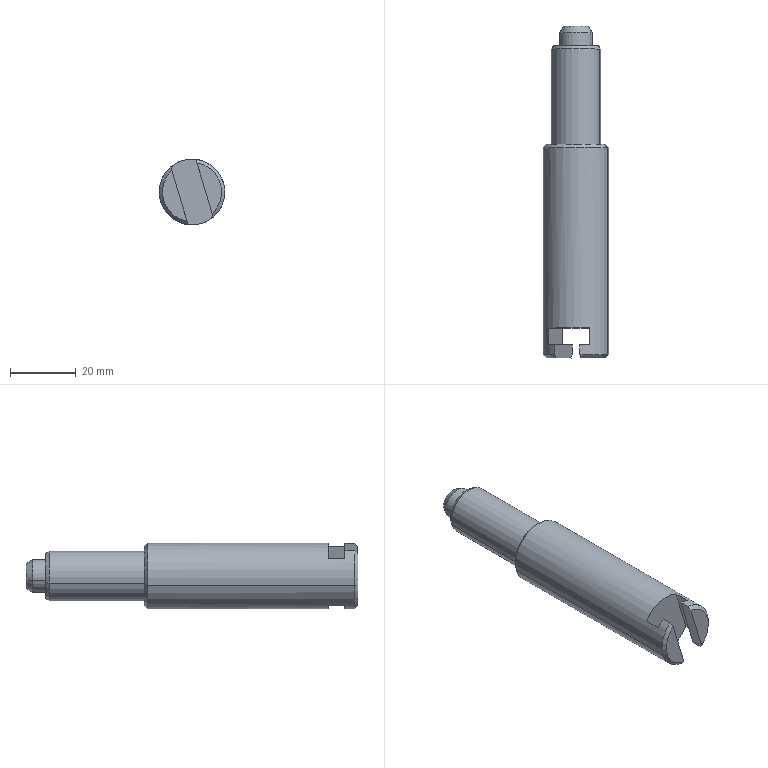Component | SolidWorks | BearingLiftingModule-1_CylinderLiftingModule-1_CHEN123-AA-27-1 | 1 solid | 27 faces | box 20 x 101 x 20 mm | volume 24230 mm3 | plane 12 | cone 9 | cylinder 6 | commonest cylinder face diameters 10 x2 15 x2 20 x2
build123d program:
from build123d import *

# Parameters (mm, degrees)
SKETCH1_R               = 10
BOSS_EXTRUDE1_DEPTH     = 65
SKETCH2_R               = 7.5
BOSS_EXTRUDE2_DEPTH     = 30
CHAMFER1_SIZE           = 1
CHAMFER1_SIZE2          = 0.5774
CHAMFER2_SIZE           = 1
CUT_EXTRUDE1_DEPTH      = 97.047
CUT_EXTRUDE1_DEPTH_BACK = 97.047
SKETCH4_R               = 5
BOSS_EXTRUDE3_DEPTH     = 6
CHAMFER3_SIZE           = 2
CHAMFER3_SIZE2          = 1.155


with BuildPart() as part:
    # Sketch1 → Boss-Extrude1 (new body)
    with BuildSketch(Plane.XY):
        Circle(SKETCH1_R)
    extrude(amount=BOSS_EXTRUDE1_DEPTH)

    # Sketch2 → Boss-Extrude2 (add)
    with BuildSketch(Plane.XY.offset(65)):
        Circle(SKETCH2_R)
    extrude(amount=BOSS_EXTRUDE2_DEPTH)

    # Chamfer1
    chamfer1_edges = [part.edges().sort_by_distance(p)[0] for p in [
        (-7.5, 0, 95),
    ]]
    chamfer1_side = [part.faces().sort_by_distance(p)[0] for p in [
        (-7.5, 0, 80),
    ]]
    chamfer(chamfer1_edges, length=CHAMFER1_SIZE, length2=CHAMFER1_SIZE2, reference=chamfer1_side[0])

    # Chamfer2
    chamfer2_edges = [part.edges().sort_by_distance(p)[0] for p in [
        (-10, 0, 0),
        (-10, 0, 65),
    ]]
    chamfer(chamfer2_edges, length=CHAMFER2_SIZE)

    # Sketch3 → Cut-Extrude1 (cut, two sides: drawn at the far end of the back side and taken through both)
    with BuildSketch(Plane(origin=(0, 0, 0), x_dir=(1, 0, 0), z_dir=(0, 1, 0)).offset(-CUT_EXTRUDE1_DEPTH_BACK)):
        Polygon((-6.6, -4), (-6.6, -9.1), (6.6, -9.1), (6.6, -4), (4, -4), (4, 0), (-4, 0), (-4, -4), align=None)
    extrude(amount=CUT_EXTRUDE1_DEPTH + CUT_EXTRUDE1_DEPTH_BACK, mode=Mode.SUBTRACT)

    # Sketch4 → Boss-Extrude3 (add)
    with BuildSketch(Plane.XY.offset(95)):
        Circle(SKETCH4_R)
    extrude(amount=BOSS_EXTRUDE3_DEPTH)

    # Chamfer3
    chamfer3_edges = [part.edges().sort_by_distance(p)[0] for p in [
        (-5, 0, 101),
    ]]
    chamfer3_side = [part.faces().sort_by_distance(p)[0] for p in [
        (-5, 0, 98),
    ]]
    chamfer(chamfer3_edges, length=CHAMFER3_SIZE, length2=CHAMFER3_SIZE2, reference=chamfer3_side[0])


solid = part.part

# Placed as in the assembly
solid = solid.moved(Location((69.999, -44.699, 30), (-90, 0, 163.304)))
STEP:
#1=COLOUR_RGB('',0.7922,0.8196,0.9333);
#2=FILL_AREA_STYLE_COLOUR('',#1);
#3=FILL_AREA_STYLE('',(#2));
#4=SURFACE_STYLE_FILL_AREA(#3);
#5=SURFACE_SIDE_STYLE('',(#4));
#6=SURFACE_STYLE_USAGE(.BOTH.,#5);
#7=PRESENTATION_STYLE_ASSIGNMENT((#6));
#8=CARTESIAN_POINT('',(2.611,2.217,1.138));
#9=VERTEX_POINT('',#8);
#10=CARTESIAN_POINT('',(2.901,2.217,1.225));
#11=VERTEX_POINT('',#10);
#12=CARTESIAN_POINT('',(2.756,2.217,1.181));
#13=DIRECTION('',(-0.,1.,-0.));
#14=DIRECTION('',(-0.9578,0.,-0.2873));
#15=AXIS2_PLACEMENT_3D('',#12,#13,#14);
#16=CIRCLE('',#15,0.1514);
#17=EDGE_CURVE('',#9,#11,#16,.T.);
#18=ORIENTED_EDGE('',*,*,#17,.F.);
#19=CARTESIAN_POINT('',(2.567,2.138,1.125));
#20=VERTEX_POINT('',#19);
#21=CARTESIAN_POINT('',(2.611,2.217,1.138));
#22=DIRECTION('',(-0.4789,-0.866,-0.1436));
#23=VECTOR('',#22,39.37);
#24=LINE('',#21,#23);
#25=EDGE_CURVE('',#9,#20,#24,.T.);
#26=ORIENTED_EDGE('',*,*,#25,.T.);
#27=CARTESIAN_POINT('',(2.944,2.138,1.238));
#28=VERTEX_POINT('',#27);
#29=CARTESIAN_POINT('',(2.756,2.138,1.181));
#30=DIRECTION('',(0.,-1.,0.));
#31=DIRECTION('',(-0.9578,0.,-0.2873));
#32=AXIS2_PLACEMENT_3D('',#29,#30,#31);
#33=CIRCLE('',#32,0.1969);
#34=EDGE_CURVE('',#28,#20,#33,.T.);
#35=ORIENTED_EDGE('',*,*,#34,.F.);
#36=CARTESIAN_POINT('',(2.901,2.217,1.225));
#37=DIRECTION('',(0.4789,-0.866,0.1436));
#38=VECTOR('',#37,39.37);
#39=LINE('',#36,#38);
#40=EDGE_CURVE('',#11,#28,#39,.T.);
#41=ORIENTED_EDGE('',*,*,#40,.F.);
#42=EDGE_LOOP('',(#18,#26,#35,#41));
#43=FACE_OUTER_BOUND('',#42,.T.);
#44=CARTESIAN_POINT('',(2.756,2.217,1.181));
#45=DIRECTION('',(0.,-1.,0.));
#46=DIRECTION('',(0.9578,0.,0.2873));
#47=AXIS2_PLACEMENT_3D('',#44,#45,#46);
#48=CONICAL_SURFACE('',#47,0.1514,0.5236);
#49=ADVANCED_FACE('',(#43),#48,.T.);
#50=ORIENTED_EDGE('',*,*,#34,.T.);
#51=CARTESIAN_POINT('',(2.567,1.98,1.125));
#52=VERTEX_POINT('',#51);
#53=CARTESIAN_POINT('',(2.567,2.217,1.125));
#54=DIRECTION('',(0.,-1.,0.));
#55=VECTOR('',#54,39.37);
#56=LINE('',#53,#55);
#57=EDGE_CURVE('',#20,#52,#56,.T.);
#58=ORIENTED_EDGE('',*,*,#57,.T.);
#59=CARTESIAN_POINT('',(2.944,1.98,1.238));
#60=VERTEX_POINT('',#59);
#61=CARTESIAN_POINT('',(2.756,1.98,1.181));
#62=DIRECTION('',(-0.,1.,-0.));
#63=DIRECTION('',(-0.9578,0.,-0.2873));
#64=AXIS2_PLACEMENT_3D('',#61,#62,#63);
#65=CIRCLE('',#64,0.1969);
#66=EDGE_CURVE('',#52,#60,#65,.T.);
#67=ORIENTED_EDGE('',*,*,#66,.T.);
#68=CARTESIAN_POINT('',(2.944,2.217,1.238));
#69=DIRECTION('',(0.,-1.,0.));
#70=VECTOR('',#69,39.37);
#71=LINE('',#68,#70);
#72=EDGE_CURVE('',#28,#60,#71,.T.);
#73=ORIENTED_EDGE('',*,*,#72,.F.);
#74=EDGE_LOOP('',(#50,#58,#67,#73));
#75=FACE_OUTER_BOUND('',#74,.T.);
#76=CARTESIAN_POINT('',(2.756,2.217,1.181));
#77=DIRECTION('',(0.,-1.,0.));
#78=DIRECTION('',(0.9578,0.,0.2873));
#79=AXIS2_PLACEMENT_3D('',#76,#77,#78);
#80=CYLINDRICAL_SURFACE('',#79,0.1969);
#81=ADVANCED_FACE('',(#75),#80,.T.);
#82=CARTESIAN_POINT('',(2.416,0.7992,1.079));
#83=VERTEX_POINT('',#82);
#84=CARTESIAN_POINT('',(3.095,0.7992,1.283));
#85=VERTEX_POINT('',#84);
#86=CARTESIAN_POINT('',(2.756,0.7992,1.181));
#87=DIRECTION('',(-0.,1.,-0.));
#88=DIRECTION('',(-0.9578,0.,-0.2873));
#89=AXIS2_PLACEMENT_3D('',#86,#87,#88);
#90=CIRCLE('',#89,0.3543);
#91=EDGE_CURVE('',#83,#85,#90,.T.);
#92=ORIENTED_EDGE('',*,*,#91,.F.);
#93=CARTESIAN_POINT('',(2.379,0.7599,1.068));
#94=VERTEX_POINT('',#93);
#95=CARTESIAN_POINT('',(2.416,0.7992,1.079));
#96=DIRECTION('',(-0.6773,-0.7071,-0.2031));
#97=VECTOR('',#96,39.37);
#98=LINE('',#95,#97);
#99=EDGE_CURVE('',#83,#94,#98,.T.);
#100=ORIENTED_EDGE('',*,*,#99,.T.);
#101=CARTESIAN_POINT('',(3.133,0.7599,1.294));
#102=VERTEX_POINT('',#101);
#103=CARTESIAN_POINT('',(2.756,0.7599,1.181));
#104=DIRECTION('',(0.,-1.,0.));
#105=DIRECTION('',(-0.9578,0.,-0.2873));
#106=AXIS2_PLACEMENT_3D('',#103,#104,#105);
#107=CIRCLE('',#106,0.3937);
#108=EDGE_CURVE('',#102,#94,#107,.T.);
#109=ORIENTED_EDGE('',*,*,#108,.F.);
#110=CARTESIAN_POINT('',(3.095,0.7992,1.283));
#111=DIRECTION('',(0.6773,-0.7071,0.2031));
#112=VECTOR('',#111,39.37);
#113=LINE('',#110,#112);
#114=EDGE_CURVE('',#85,#102,#113,.T.);
#115=ORIENTED_EDGE('',*,*,#114,.F.);
#116=EDGE_LOOP('',(#92,#100,#109,#115));
#117=FACE_OUTER_BOUND('',#116,.T.);
#118=CARTESIAN_POINT('',(2.756,0.7992,1.181));
#119=DIRECTION('',(0.,-1.,0.));
#120=DIRECTION('',(0.9578,0.,0.2873));
#121=AXIS2_PLACEMENT_3D('',#118,#119,#120);
#122=CONICAL_SURFACE('',#121,0.3543,0.7854);
#123=ADVANCED_FACE('',(#117),#122,.T.);
#124=CARTESIAN_POINT('',(2.416,-1.76,1.079));
#125=VERTEX_POINT('',#124);
#126=CARTESIAN_POINT('',(2.696,-1.76,0.8318));
#127=VERTEX_POINT('',#126);
#128=CARTESIAN_POINT('',(2.756,-1.76,1.181));
#129=DIRECTION('',(0.,-1.,0.));
#130=DIRECTION('',(-0.9578,0.,-0.2873));
#131=AXIS2_PLACEMENT_3D('',#128,#129,#130);
#132=CIRCLE('',#131,0.3543);
#133=EDGE_CURVE('',#125,#127,#132,.T.);
#134=ORIENTED_EDGE('',*,*,#133,.F.);
#135=CARTESIAN_POINT('',(2.379,-1.72,1.068));
#136=VERTEX_POINT('',#135);
#137=CARTESIAN_POINT('',(2.379,-1.72,1.068));
#138=DIRECTION('',(-0.6773,0.7071,-0.2031));
#139=VECTOR('',#138,39.37);
#140=LINE('',#137,#139);
#141=EDGE_CURVE('',#125,#136,#140,.T.);
#142=ORIENTED_EDGE('',*,*,#141,.T.);
#143=CARTESIAN_POINT('',(2.709,-1.72,0.7902));
#144=VERTEX_POINT('',#143);
#145=CARTESIAN_POINT('',(2.756,-1.72,1.181));
#146=DIRECTION('',(-0.,1.,-0.));
#147=DIRECTION('',(-0.9578,0.,-0.2873));
#148=AXIS2_PLACEMENT_3D('',#145,#146,#147);
#149=CIRCLE('',#148,0.3937);
#150=EDGE_CURVE('',#144,#136,#149,.T.);
#151=ORIENTED_EDGE('',*,*,#150,.F.);
#152=CARTESIAN_POINT('',(2.696,-1.76,0.8318));
#153=CARTESIAN_POINT('',(2.7,-1.747,0.8179));
#154=CARTESIAN_POINT('',(2.705,-1.734,0.804));
#155=CARTESIAN_POINT('',(2.709,-1.72,0.7902));
#156=B_SPLINE_CURVE_WITH_KNOTS('',3,(#152,#153,#154,#155),.UNSPECIFIED.,.F.,.F.,(4,4),(0.03786,0.03933),.UNSPECIFIED.);
#157=EDGE_CURVE('',#127,#144,#156,.T.);
#158=ORIENTED_EDGE('',*,*,#157,.F.);
#159=EDGE_LOOP('',(#134,#142,#151,#158));
#160=FACE_OUTER_BOUND('',#159,.T.);
#161=CARTESIAN_POINT('',(2.756,-1.72,1.181));
#162=DIRECTION('',(-0.,1.,-0.));
#163=DIRECTION('',(-0.9578,0.,-0.2873));
#164=AXIS2_PLACEMENT_3D('',#161,#162,#163);
#165=CONICAL_SURFACE('',#164,0.3937,0.7854);
#166=ADVANCED_FACE('',(#160),#165,.T.);
#167=CARTESIAN_POINT('',(2.495,1.98,1.103));
#168=VERTEX_POINT('',#167);
#169=CARTESIAN_POINT('',(3.017,1.98,1.259));
#170=VERTEX_POINT('',#169);
#171=CARTESIAN_POINT('',(2.756,1.98,1.181));
#172=DIRECTION('',(-0.,1.,-0.));
#173=DIRECTION('',(-0.9578,0.,-0.2873));
#174=AXIS2_PLACEMENT_3D('',#171,#172,#173);
#175=CIRCLE('',#174,0.2725);
#176=EDGE_CURVE('',#168,#170,#175,.T.);
#177=ORIENTED_EDGE('',*,*,#176,.F.);
#178=CARTESIAN_POINT('',(2.473,1.941,1.096));
#179=VERTEX_POINT('',#178);
#180=CARTESIAN_POINT('',(2.495,1.98,1.103));
#181=DIRECTION('',(-0.4789,-0.866,-0.1436));
#182=VECTOR('',#181,39.37);
#183=LINE('',#180,#182);
#184=EDGE_CURVE('',#168,#179,#183,.T.);
#185=ORIENTED_EDGE('',*,*,#184,.T.);
#186=CARTESIAN_POINT('',(3.039,1.941,1.266));
#187=VERTEX_POINT('',#186);
#188=CARTESIAN_POINT('',(2.756,1.941,1.181));
#189=DIRECTION('',(0.,-1.,0.));
#190=DIRECTION('',(-0.9578,0.,-0.2873));
#191=AXIS2_PLACEMENT_3D('',#188,#189,#190);
#192=CIRCLE('',#191,0.2953);
#193=EDGE_CURVE('',#187,#179,#192,.T.);
#194=ORIENTED_EDGE('',*,*,#193,.F.);
#195=CARTESIAN_POINT('',(3.017,1.98,1.259));
#196=DIRECTION('',(0.4789,-0.866,0.1436));
#197=VECTOR('',#196,39.37);
#198=LINE('',#195,#197);
#199=EDGE_CURVE('',#170,#187,#198,.T.);
#200=ORIENTED_EDGE('',*,*,#199,.F.);
#201=EDGE_LOOP('',(#177,#185,#194,#200));
#202=FACE_OUTER_BOUND('',#201,.T.);
#203=CARTESIAN_POINT('',(2.756,1.98,1.181));
#204=DIRECTION('',(0.,-1.,0.));
#205=DIRECTION('',(0.9578,0.,0.2873));
#206=AXIS2_PLACEMENT_3D('',#203,#204,#205);
#207=CONICAL_SURFACE('',#206,0.2725,0.5236);
#208=ADVANCED_FACE('',(#202),#207,.T.);
#209=ORIENTED_EDGE('',*,*,#193,.T.);
#210=CARTESIAN_POINT('',(2.473,0.7992,1.096));
#211=VERTEX_POINT('',#210);
#212=CARTESIAN_POINT('',(2.473,1.98,1.096));
#213=DIRECTION('',(0.,-1.,0.));
#214=VECTOR('',#213,39.37);
#215=LINE('',#212,#214);
#216=EDGE_CURVE('',#179,#211,#215,.T.);
#217=ORIENTED_EDGE('',*,*,#216,.T.);
#218=CARTESIAN_POINT('',(3.039,0.7992,1.266));
#219=VERTEX_POINT('',#218);
#220=CARTESIAN_POINT('',(2.756,0.7992,1.181));
#221=DIRECTION('',(-0.,1.,-0.));
#222=DIRECTION('',(-0.9578,0.,-0.2873));
#223=AXIS2_PLACEMENT_3D('',#220,#221,#222);
#224=CIRCLE('',#223,0.2953);
#225=EDGE_CURVE('',#211,#219,#224,.T.);
#226=ORIENTED_EDGE('',*,*,#225,.T.);
#227=CARTESIAN_POINT('',(3.039,1.98,1.266));
#228=DIRECTION('',(0.,-1.,0.));
#229=VECTOR('',#228,39.37);
#230=LINE('',#227,#229);
#231=EDGE_CURVE('',#187,#219,#230,.T.);
#232=ORIENTED_EDGE('',*,*,#231,.F.);
#233=EDGE_LOOP('',(#209,#217,#226,#232));
#234=FACE_OUTER_BOUND('',#233,.T.);
#235=CARTESIAN_POINT('',(2.756,1.98,1.181));
#236=DIRECTION('',(0.,-1.,0.));
#237=DIRECTION('',(0.9578,0.,0.2873));
#238=AXIS2_PLACEMENT_3D('',#235,#236,#237);
#239=CYLINDRICAL_SURFACE('',#238,0.2953);
#240=ADVANCED_FACE('',(#234),#239,.T.);
#241=ORIENTED_EDGE('',*,*,#108,.T.);
#242=CARTESIAN_POINT('',(2.379,0.7992,1.068));
#243=DIRECTION('',(0.,-1.,0.));
#244=VECTOR('',#243,39.37);
#245=LINE('',#242,#244);
#246=EDGE_CURVE('',#94,#136,#245,.T.);
#247=ORIENTED_EDGE('',*,*,#246,.T.);
#248=CARTESIAN_POINT('',(2.501,-1.72,1.481));
#249=VERTEX_POINT('',#248);
#250=CARTESIAN_POINT('',(2.756,-1.72,1.181));
#251=DIRECTION('',(-0.,1.,-0.));
#252=DIRECTION('',(-0.9578,0.,-0.2873));
#253=AXIS2_PLACEMENT_3D('',#250,#251,#252);
#254=CIRCLE('',#253,0.3937);
#255=EDGE_CURVE('',#136,#249,#254,.T.);
#256=ORIENTED_EDGE('',*,*,#255,.T.);
#257=CARTESIAN_POINT('',(2.501,-1.602,1.481));
#258=VERTEX_POINT('',#257);
#259=CARTESIAN_POINT('',(2.501,0.7992,1.481));
#260=DIRECTION('',(-0.,1.,-0.));
#261=VECTOR('',#260,39.37);
#262=LINE('',#259,#261);
#263=EDGE_CURVE('',#249,#258,#262,.T.);
#264=ORIENTED_EDGE('',*,*,#263,.T.);
#265=CARTESIAN_POINT('',(2.422,-1.602,1.39));
#266=VERTEX_POINT('',#265);
#267=CARTESIAN_POINT('',(2.756,-1.602,1.181));
#268=DIRECTION('',(0.,-1.,0.));
#269=DIRECTION('',(0.9578,0.,0.2873));
#270=AXIS2_PLACEMENT_3D('',#267,#268,#269);
#271=CIRCLE('',#270,0.3937);
#272=EDGE_CURVE('',#258,#266,#271,.T.);
#273=ORIENTED_EDGE('',*,*,#272,.T.);
#274=CARTESIAN_POINT('',(2.422,-1.402,1.39));
#275=VERTEX_POINT('',#274);
#276=CARTESIAN_POINT('',(2.422,0.7992,1.39));
#277=DIRECTION('',(-0.,1.,-0.));
#278=VECTOR('',#277,39.37);
#279=LINE('',#276,#278);
#280=EDGE_CURVE('',#266,#275,#279,.T.);
#281=ORIENTED_EDGE('',*,*,#280,.T.);
#282=CARTESIAN_POINT('',(2.92,-1.402,1.539));
#283=VERTEX_POINT('',#282);
#284=CARTESIAN_POINT('',(2.756,-1.402,1.181));
#285=DIRECTION('',(-0.,1.,-0.));
#286=DIRECTION('',(-0.9578,0.,-0.2873));
#287=AXIS2_PLACEMENT_3D('',#284,#285,#286);
#288=CIRCLE('',#287,0.3937);
#289=EDGE_CURVE('',#275,#283,#288,.T.);
#290=ORIENTED_EDGE('',*,*,#289,.T.);
#291=CARTESIAN_POINT('',(2.92,-1.602,1.539));
#292=VERTEX_POINT('',#291);
#293=CARTESIAN_POINT('',(2.92,0.7992,1.539));
#294=DIRECTION('',(0.,-1.,0.));
#295=VECTOR('',#294,39.37);
#296=LINE('',#293,#295);
#297=EDGE_CURVE('',#283,#292,#296,.T.);
#298=ORIENTED_EDGE('',*,*,#297,.T.);
#299=CARTESIAN_POINT('',(2.803,-1.602,1.572));
#300=VERTEX_POINT('',#299);
#301=CARTESIAN_POINT('',(2.756,-1.602,1.181));
#302=DIRECTION('',(0.,-1.,0.));
#303=DIRECTION('',(0.9578,0.,0.2873));
#304=AXIS2_PLACEMENT_3D('',#301,#302,#303);
#305=CIRCLE('',#304,0.3937);
#306=EDGE_CURVE('',#292,#300,#305,.T.);
#307=ORIENTED_EDGE('',*,*,#306,.T.);
#308=CARTESIAN_POINT('',(2.803,-1.72,1.572));
#309=VERTEX_POINT('',#308);
#310=CARTESIAN_POINT('',(2.803,0.7992,1.572));
#311=DIRECTION('',(0.,-1.,0.));
#312=VECTOR('',#311,39.37);
#313=LINE('',#310,#312);
#314=EDGE_CURVE('',#300,#309,#313,.T.);
#315=ORIENTED_EDGE('',*,*,#314,.T.);
#316=CARTESIAN_POINT('',(3.133,-1.72,1.294));
#317=VERTEX_POINT('',#316);
#318=CARTESIAN_POINT('',(2.756,-1.72,1.181));
#319=DIRECTION('',(-0.,1.,-0.));
#320=DIRECTION('',(-0.9578,0.,-0.2873));
#321=AXIS2_PLACEMENT_3D('',#318,#319,#320);
#322=CIRCLE('',#321,0.3937);
#323=EDGE_CURVE('',#309,#317,#322,.T.);
#324=ORIENTED_EDGE('',*,*,#323,.T.);
#325=CARTESIAN_POINT('',(3.133,0.7992,1.294));
#326=DIRECTION('',(0.,-1.,0.));
#327=VECTOR('',#326,39.37);
#328=LINE('',#325,#327);
#329=EDGE_CURVE('',#102,#317,#328,.T.);
#330=ORIENTED_EDGE('',*,*,#329,.F.);
#331=EDGE_LOOP('',(#241,#247,#256,#264,#273,#281,#290,#298,#307,#315,#324,#330));
#332=FACE_OUTER_BOUND('',#331,.T.);
#333=CARTESIAN_POINT('',(2.756,0.7992,1.181));
#334=DIRECTION('',(0.,-1.,0.));
#335=DIRECTION('',(0.9578,0.,0.2873));
#336=AXIS2_PLACEMENT_3D('',#333,#334,#335);
#337=CYLINDRICAL_SURFACE('',#336,0.3937);
#338=ADVANCED_FACE('',(#332),#337,.T.);
#339=CARTESIAN_POINT('',(2.998,-1.76,0.9223));
#340=VERTEX_POINT('',#339);
#341=CARTESIAN_POINT('',(2.816,-1.76,1.53));
#342=VERTEX_POINT('',#341);
#343=CARTESIAN_POINT('',(2.756,-1.76,1.181));
#344=DIRECTION('',(0.,-1.,0.));
#345=DIRECTION('',(-0.9578,0.,-0.2873));
#346=AXIS2_PLACEMENT_3D('',#343,#344,#345);
#347=CIRCLE('',#346,0.3543);
#348=EDGE_CURVE('',#340,#342,#347,.T.);
#349=ORIENTED_EDGE('',*,*,#348,.T.);
#350=CARTESIAN_POINT('',(3.02,-1.76,0.8492));
#351=DIRECTION('',(-0.2873,0.,0.9578));
#352=VECTOR('',#351,39.37);
#353=LINE('',#350,#352);
#354=EDGE_CURVE('',#340,#342,#353,.T.);
#355=ORIENTED_EDGE('',*,*,#354,.F.);
#356=EDGE_LOOP('',(#349,#355));
#357=FACE_OUTER_BOUND('',#356,.T.);
#358=CARTESIAN_POINT('',(2.756,-1.76,1.181));
#359=DIRECTION('',(-0.,1.,-0.));
#360=DIRECTION('',(-0.9578,-0.,-0.2873));
#361=AXIS2_PLACEMENT_3D('',#358,#359,#360);
#362=PLANE('',#361);
#363=ADVANCED_FACE('',(#357),#362,.F.);
#364=CARTESIAN_POINT('',(3.01,-1.72,0.8807));
#365=VERTEX_POINT('',#364);
#366=CARTESIAN_POINT('',(3.01,-1.72,0.8807));
#367=CARTESIAN_POINT('',(3.006,-1.734,0.8945));
#368=CARTESIAN_POINT('',(3.002,-1.747,0.9084));
#369=CARTESIAN_POINT('',(2.998,-1.76,0.9223));
#370=B_SPLINE_CURVE_WITH_KNOTS('',3,(#366,#367,#368,#369),.UNSPECIFIED.,.F.,.F.,(4,4),(0.01732,0.01881),.UNSPECIFIED.);
#371=EDGE_CURVE('',#365,#340,#370,.T.);
#372=ORIENTED_EDGE('',*,*,#371,.F.);
#373=CARTESIAN_POINT('',(2.756,-1.72,1.181));
#374=DIRECTION('',(-0.,1.,-0.));
#375=DIRECTION('',(-0.9578,0.,-0.2873));
#376=AXIS2_PLACEMENT_3D('',#373,#374,#375);
#377=CIRCLE('',#376,0.3937);
#378=EDGE_CURVE('',#317,#365,#377,.T.);
#379=ORIENTED_EDGE('',*,*,#378,.F.);
#380=ORIENTED_EDGE('',*,*,#323,.F.);
#381=CARTESIAN_POINT('',(2.816,-1.76,1.53));
#382=CARTESIAN_POINT('',(2.811,-1.747,1.544));
#383=CARTESIAN_POINT('',(2.807,-1.734,1.558));
#384=CARTESIAN_POINT('',(2.803,-1.72,1.572));
#385=B_SPLINE_CURVE_WITH_KNOTS('',3,(#381,#382,#383,#384),.UNSPECIFIED.,.F.,.F.,(4,4),(0.03786,0.03933),.UNSPECIFIED.);
#386=EDGE_CURVE('',#342,#309,#385,.T.);
#387=ORIENTED_EDGE('',*,*,#386,.F.);
#388=ORIENTED_EDGE('',*,*,#348,.F.);
#389=EDGE_LOOP('',(#372,#379,#380,#387,#388));
#390=FACE_OUTER_BOUND('',#389,.T.);
#391=CARTESIAN_POINT('',(2.756,-1.72,1.181));
#392=DIRECTION('',(-0.,1.,-0.));
#393=DIRECTION('',(-0.9578,0.,-0.2873));
#394=AXIS2_PLACEMENT_3D('',#391,#392,#393);
#395=CONICAL_SURFACE('',#394,0.3937,0.7854);
#396=ADVANCED_FACE('',(#390),#395,.T.);
#397=ORIENTED_EDGE('',*,*,#246,.F.);
#398=CARTESIAN_POINT('',(2.756,0.7599,1.181));
#399=DIRECTION('',(0.,-1.,0.));
#400=DIRECTION('',(-0.9578,0.,-0.2873));
#401=AXIS2_PLACEMENT_3D('',#398,#399,#400);
#402=CIRCLE('',#401,0.3937);
#403=EDGE_CURVE('',#94,#102,#402,.T.);
#404=ORIENTED_EDGE('',*,*,#403,.T.);
#405=ORIENTED_EDGE('',*,*,#329,.T.);
#406=ORIENTED_EDGE('',*,*,#378,.T.);
#407=CARTESIAN_POINT('',(3.01,-1.602,0.8807));
#408=VERTEX_POINT('',#407);
#409=CARTESIAN_POINT('',(3.01,0.7992,0.8807));
#410=DIRECTION('',(-0.,1.,-0.));
#411=VECTOR('',#410,39.37);
#412=LINE('',#409,#411);
#413=EDGE_CURVE('',#365,#408,#412,.T.);
#414=ORIENTED_EDGE('',*,*,#413,.T.);
#415=CARTESIAN_POINT('',(3.09,-1.602,0.9724));
#416=VERTEX_POINT('',#415);
#417=CARTESIAN_POINT('',(2.756,-1.602,1.181));
#418=DIRECTION('',(0.,-1.,0.));
#419=DIRECTION('',(0.9578,0.,0.2873));
#420=AXIS2_PLACEMENT_3D('',#417,#418,#419);
#421=CIRCLE('',#420,0.3937);
#422=EDGE_CURVE('',#408,#416,#421,.T.);
#423=ORIENTED_EDGE('',*,*,#422,.T.);
#424=CARTESIAN_POINT('',(3.09,-1.402,0.9724));
#425=VERTEX_POINT('',#424);
#426=CARTESIAN_POINT('',(3.09,0.7992,0.9724));
#427=DIRECTION('',(-0.,1.,-0.));
#428=VECTOR('',#427,39.37);
#429=LINE('',#426,#428);
#430=EDGE_CURVE('',#416,#425,#429,.T.);
#431=ORIENTED_EDGE('',*,*,#430,.T.);
#432=CARTESIAN_POINT('',(2.592,-1.402,0.8231));
#433=VERTEX_POINT('',#432);
#434=CARTESIAN_POINT('',(2.756,-1.402,1.181));
#435=DIRECTION('',(-0.,1.,-0.));
#436=DIRECTION('',(-0.9578,0.,-0.2873));
#437=AXIS2_PLACEMENT_3D('',#434,#435,#436);
#438=CIRCLE('',#437,0.3937);
#439=EDGE_CURVE('',#425,#433,#438,.T.);
#440=ORIENTED_EDGE('',*,*,#439,.T.);
#441=CARTESIAN_POINT('',(2.592,-1.602,0.8231));
#442=VERTEX_POINT('',#441);
#443=CARTESIAN_POINT('',(2.592,0.7992,0.8231));
#444=DIRECTION('',(0.,-1.,0.));
#445=VECTOR('',#444,39.37);
#446=LINE('',#443,#445);
#447=EDGE_CURVE('',#433,#442,#446,.T.);
#448=ORIENTED_EDGE('',*,*,#447,.T.);
#449=CARTESIAN_POINT('',(2.709,-1.602,0.7902));
#450=VERTEX_POINT('',#449);
#451=CARTESIAN_POINT('',(2.756,-1.602,1.181));
#452=DIRECTION('',(0.,-1.,0.));
#453=DIRECTION('',(0.9578,0.,0.2873));
#454=AXIS2_PLACEMENT_3D('',#451,#452,#453);
#455=CIRCLE('',#454,0.3937);
#456=EDGE_CURVE('',#442,#450,#455,.T.);
#457=ORIENTED_EDGE('',*,*,#456,.T.);
#458=CARTESIAN_POINT('',(2.709,0.7992,0.7902));
#459=DIRECTION('',(0.,-1.,0.));
#460=VECTOR('',#459,39.37);
#461=LINE('',#458,#460);
#462=EDGE_CURVE('',#450,#144,#461,.T.);
#463=ORIENTED_EDGE('',*,*,#462,.T.);
#464=ORIENTED_EDGE('',*,*,#150,.T.);
#465=EDGE_LOOP('',(#397,#404,#405,#406,#414,#423,#431,#440,#448,#457,#463,#464));
#466=FACE_OUTER_BOUND('',#465,.T.);
#467=CARTESIAN_POINT('',(2.756,0.7992,1.181));
#468=DIRECTION('',(0.,-1.,0.));
#469=DIRECTION('',(0.9578,0.,0.2873));
#470=AXIS2_PLACEMENT_3D('',#467,#468,#469);
#471=CYLINDRICAL_SURFACE('',#470,0.3937);
#472=ADVANCED_FACE('',(#466),#471,.T.);
#473=CARTESIAN_POINT('',(2.756,0.7992,1.181));
#474=DIRECTION('',(-0.,1.,-0.));
#475=DIRECTION('',(-0.9578,0.,-0.2873));
#476=AXIS2_PLACEMENT_3D('',#473,#474,#475);
#477=CIRCLE('',#476,0.3543);
#478=EDGE_CURVE('',#85,#83,#477,.T.);
#479=ORIENTED_EDGE('',*,*,#478,.T.);
#480=ORIENTED_EDGE('',*,*,#91,.T.);
#481=EDGE_LOOP('',(#479,#480));
#482=FACE_OUTER_BOUND('',#481,.T.);
#483=CARTESIAN_POINT('',(2.756,0.7992,1.181));
#484=DIRECTION('',(-0.,1.,-0.));
#485=DIRECTION('',(-0.9578,0.,-0.2873));
#486=AXIS2_PLACEMENT_3D('',#483,#484,#485);
#487=CIRCLE('',#486,0.2953);
#488=EDGE_CURVE('',#219,#211,#487,.T.);
#489=ORIENTED_EDGE('',*,*,#488,.F.);
#490=ORIENTED_EDGE('',*,*,#225,.F.);
#491=EDGE_LOOP('',(#489,#490));
#492=FACE_BOUND('',#491,.T.);
#493=CARTESIAN_POINT('',(2.756,0.7992,1.181));
#494=DIRECTION('',(-0.,1.,-0.));
#495=DIRECTION('',(-0.9578,-0.,-0.2873));
#496=AXIS2_PLACEMENT_3D('',#493,#494,#495);
#497=PLANE('',#496);
#498=ADVANCED_FACE('',(#482,#492),#497,.T.);
#499=CARTESIAN_POINT('',(2.514,-1.76,1.44));
#500=VERTEX_POINT('',#499);
#501=CARTESIAN_POINT('',(2.756,-1.76,1.181));
#502=DIRECTION('',(0.,-1.,0.));
#503=DIRECTION('',(-0.9578,0.,-0.2873));
#504=AXIS2_PLACEMENT_3D('',#501,#502,#503);
#505=CIRCLE('',#504,0.3543);
#506=EDGE_CURVE('',#500,#125,#505,.T.);
#507=ORIENTED_EDGE('',*,*,#506,.T.);
#508=ORIENTED_EDGE('',*,*,#133,.T.);
#509=CARTESIAN_POINT('',(2.718,-1.76,0.7588));
#510=DIRECTION('',(-0.2873,0.,0.9578));
#511=VECTOR('',#510,39.37);
#512=LINE('',#509,#511);
#513=EDGE_CURVE('',#127,#500,#512,.T.);
#514=ORIENTED_EDGE('',*,*,#513,.T.);
#515=EDGE_LOOP('',(#507,#508,#514));
#516=FACE_OUTER_BOUND('',#515,.T.);
#517=CARTESIAN_POINT('',(2.756,-1.76,1.181));
#518=DIRECTION('',(-0.,1.,-0.));
#519=DIRECTION('',(-0.9578,-0.,-0.2873));
#520=AXIS2_PLACEMENT_3D('',#517,#518,#519);
#521=PLANE('',#520);
#522=ADVANCED_FACE('',(#516),#521,.F.);
#523=ORIENTED_EDGE('',*,*,#216,.F.);
#524=CARTESIAN_POINT('',(2.756,1.941,1.181));
#525=DIRECTION('',(0.,-1.,0.));
#526=DIRECTION('',(-0.9578,0.,-0.2873));
#527=AXIS2_PLACEMENT_3D('',#524,#525,#526);
#528=CIRCLE('',#527,0.2953);
#529=EDGE_CURVE('',#179,#187,#528,.T.);
#530=ORIENTED_EDGE('',*,*,#529,.T.);
#531=ORIENTED_EDGE('',*,*,#231,.T.);
#532=ORIENTED_EDGE('',*,*,#488,.T.);
#533=EDGE_LOOP('',(#523,#530,#531,#532));
#534=FACE_OUTER_BOUND('',#533,.T.);
#535=CARTESIAN_POINT('',(2.756,1.98,1.181));
#536=DIRECTION('',(0.,-1.,0.));
#537=DIRECTION('',(0.9578,0.,0.2873));
#538=AXIS2_PLACEMENT_3D('',#535,#536,#537);
#539=CYLINDRICAL_SURFACE('',#538,0.2953);
#540=ADVANCED_FACE('',(#534),#539,.T.);
#541=CARTESIAN_POINT('',(2.756,1.98,1.181));
#542=DIRECTION('',(-0.,1.,-0.));
#543=DIRECTION('',(-0.9578,0.,-0.2873));
#544=AXIS2_PLACEMENT_3D('',#541,#542,#543);
#545=CIRCLE('',#544,0.1969);
#546=EDGE_CURVE('',#60,#52,#545,.T.);
#547=ORIENTED_EDGE('',*,*,#546,.F.);
#548=ORIENTED_EDGE('',*,*,#66,.F.);
#549=EDGE_LOOP('',(#547,#548));
#550=FACE_BOUND('',#549,.T.);
#551=CARTESIAN_POINT('',(2.756,1.98,1.181));
#552=DIRECTION('',(-0.,1.,-0.));
#553=DIRECTION('',(-0.9578,0.,-0.2873));
#554=AXIS2_PLACEMENT_3D('',#551,#552,#553);
#555=CIRCLE('',#554,0.2725);
#556=EDGE_CURVE('',#170,#168,#555,.T.);
#557=ORIENTED_EDGE('',*,*,#556,.T.);
#558=ORIENTED_EDGE('',*,*,#176,.T.);
#559=EDGE_LOOP('',(#557,#558));
#560=FACE_OUTER_BOUND('',#559,.T.);
#561=CARTESIAN_POINT('',(2.756,1.98,1.181));
#562=DIRECTION('',(-0.,1.,-0.));
#563=DIRECTION('',(-0.9578,-0.,-0.2873));
#564=AXIS2_PLACEMENT_3D('',#561,#562,#563);
#565=PLANE('',#564);
#566=ADVANCED_FACE('',(#550,#560),#565,.T.);
#567=ORIENTED_EDGE('',*,*,#184,.F.);
#568=ORIENTED_EDGE('',*,*,#556,.F.);
#569=ORIENTED_EDGE('',*,*,#199,.T.);
#570=ORIENTED_EDGE('',*,*,#529,.F.);
#571=EDGE_LOOP('',(#567,#568,#569,#570));
#572=FACE_OUTER_BOUND('',#571,.T.);
#573=CARTESIAN_POINT('',(2.756,1.98,1.181));
#574=DIRECTION('',(0.,-1.,0.));
#575=DIRECTION('',(0.9578,0.,0.2873));
#576=AXIS2_PLACEMENT_3D('',#573,#574,#575);
#577=CONICAL_SURFACE('',#576,0.2725,0.5236);
#578=ADVANCED_FACE('',(#572),#577,.T.);
#579=ORIENTED_EDGE('',*,*,#141,.F.);
#580=ORIENTED_EDGE('',*,*,#506,.F.);
#581=CARTESIAN_POINT('',(2.501,-1.72,1.481));
#582=CARTESIAN_POINT('',(2.506,-1.734,1.468));
#583=CARTESIAN_POINT('',(2.51,-1.747,1.454));
#584=CARTESIAN_POINT('',(2.514,-1.76,1.44));
#585=B_SPLINE_CURVE_WITH_KNOTS('',3,(#581,#582,#583,#584),.UNSPECIFIED.,.F.,.F.,(4,4),(0.01732,0.01881),.UNSPECIFIED.);
#586=EDGE_CURVE('',#249,#500,#585,.T.);
#587=ORIENTED_EDGE('',*,*,#586,.F.);
#588=ORIENTED_EDGE('',*,*,#255,.F.);
#589=EDGE_LOOP('',(#579,#580,#587,#588));
#590=FACE_OUTER_BOUND('',#589,.T.);
#591=CARTESIAN_POINT('',(2.756,-1.72,1.181));
#592=DIRECTION('',(-0.,1.,-0.));
#593=DIRECTION('',(-0.9578,0.,-0.2873));
#594=AXIS2_PLACEMENT_3D('',#591,#592,#593);
#595=CONICAL_SURFACE('',#594,0.3937,0.7854);
#596=ADVANCED_FACE('',(#590),#595,.T.);
#597=ORIENTED_EDGE('',*,*,#99,.F.);
#598=ORIENTED_EDGE('',*,*,#478,.F.);
#599=ORIENTED_EDGE('',*,*,#114,.T.);
#600=ORIENTED_EDGE('',*,*,#403,.F.);
#601=EDGE_LOOP('',(#597,#598,#599,#600));
#602=FACE_OUTER_BOUND('',#601,.T.);
#603=CARTESIAN_POINT('',(2.756,0.7992,1.181));
#604=DIRECTION('',(0.,-1.,0.));
#605=DIRECTION('',(0.9578,0.,0.2873));
#606=AXIS2_PLACEMENT_3D('',#603,#604,#605);
#607=CONICAL_SURFACE('',#606,0.3543,0.7854);
#608=ADVANCED_FACE('',(#602),#607,.T.);
#609=CARTESIAN_POINT('',(2.62,-1.402,0.7293));
#610=DIRECTION('',(-0.2873,0.,0.9578));
#611=VECTOR('',#610,39.37);
#612=LINE('',#609,#611);
#613=EDGE_CURVE('',#433,#275,#612,.T.);
#614=ORIENTED_EDGE('',*,*,#613,.F.);
#615=ORIENTED_EDGE('',*,*,#439,.F.);
#616=CARTESIAN_POINT('',(3.118,-1.402,0.8787));
#617=DIRECTION('',(-0.2873,0.,0.9578));
#618=VECTOR('',#617,39.37);
#619=LINE('',#616,#618);
#620=EDGE_CURVE('',#425,#283,#619,.T.);
#621=ORIENTED_EDGE('',*,*,#620,.T.);
#622=ORIENTED_EDGE('',*,*,#289,.F.);
#623=EDGE_LOOP('',(#614,#615,#621,#622));
#624=FACE_OUTER_BOUND('',#623,.T.);
#625=CARTESIAN_POINT('',(3.118,-1.402,0.8787));
#626=DIRECTION('',(-0.,1.,-0.));
#627=DIRECTION('',(-0.9578,-0.,-0.2873));
#628=AXIS2_PLACEMENT_3D('',#625,#626,#627);
#629=PLANE('',#628);
#630=ADVANCED_FACE('',(#624),#629,.F.);
#631=ORIENTED_EDGE('',*,*,#620,.F.);
#632=ORIENTED_EDGE('',*,*,#430,.F.);
#633=CARTESIAN_POINT('',(3.118,-1.602,0.8787));
#634=DIRECTION('',(-0.2873,0.,0.9578));
#635=VECTOR('',#634,39.37);
#636=LINE('',#633,#635);
#637=EDGE_CURVE('',#416,#292,#636,.T.);
#638=ORIENTED_EDGE('',*,*,#637,.T.);
#639=ORIENTED_EDGE('',*,*,#297,.F.);
#640=EDGE_LOOP('',(#631,#632,#638,#639));
#641=FACE_OUTER_BOUND('',#640,.T.);
#642=CARTESIAN_POINT('',(3.118,-1.602,0.8787));
#643=DIRECTION('',(0.9578,0.,0.2873));
#644=DIRECTION('',(-0.,1.,-0.));
#645=AXIS2_PLACEMENT_3D('',#642,#643,#644);
#646=PLANE('',#645);
#647=ADVANCED_FACE('',(#641),#646,.F.);
#648=ORIENTED_EDGE('',*,*,#637,.F.);
#649=ORIENTED_EDGE('',*,*,#422,.F.);
#650=CARTESIAN_POINT('',(3.02,-1.602,0.8492));
#651=DIRECTION('',(-0.2873,0.,0.9578));
#652=VECTOR('',#651,39.37);
#653=LINE('',#650,#652);
#654=EDGE_CURVE('',#408,#300,#653,.T.);
#655=ORIENTED_EDGE('',*,*,#654,.T.);
#656=ORIENTED_EDGE('',*,*,#306,.F.);
#657=EDGE_LOOP('',(#648,#649,#655,#656));
#658=FACE_OUTER_BOUND('',#657,.T.);
#659=CARTESIAN_POINT('',(3.118,-1.602,0.8787));
#660=DIRECTION('',(0.,-1.,0.));
#661=DIRECTION('',(0.9578,0.,0.2873));
#662=AXIS2_PLACEMENT_3D('',#659,#660,#661);
#663=PLANE('',#662);
#664=ADVANCED_FACE('',(#658),#663,.F.);
#665=CARTESIAN_POINT('',(2.718,-1.602,0.7588));
#666=DIRECTION('',(-0.2873,0.,0.9578));
#667=VECTOR('',#666,39.37);
#668=LINE('',#665,#667);
#669=EDGE_CURVE('',#450,#258,#668,.T.);
#670=ORIENTED_EDGE('',*,*,#669,.F.);
#671=ORIENTED_EDGE('',*,*,#456,.F.);
#672=CARTESIAN_POINT('',(2.62,-1.602,0.7293));
#673=DIRECTION('',(-0.2873,0.,0.9578));
#674=VECTOR('',#673,39.37);
#675=LINE('',#672,#674);
#676=EDGE_CURVE('',#442,#266,#675,.T.);
#677=ORIENTED_EDGE('',*,*,#676,.T.);
#678=ORIENTED_EDGE('',*,*,#272,.F.);
#679=EDGE_LOOP('',(#670,#671,#677,#678));
#680=FACE_OUTER_BOUND('',#679,.T.);
#681=CARTESIAN_POINT('',(2.62,-1.602,0.7293));
#682=DIRECTION('',(0.,-1.,0.));
#683=DIRECTION('',(0.9578,0.,0.2873));
#684=AXIS2_PLACEMENT_3D('',#681,#682,#683);
#685=PLANE('',#684);
#686=ADVANCED_FACE('',(#680),#685,.F.);
#687=ORIENTED_EDGE('',*,*,#613,.T.);
#688=ORIENTED_EDGE('',*,*,#280,.F.);
#689=ORIENTED_EDGE('',*,*,#676,.F.);
#690=ORIENTED_EDGE('',*,*,#447,.F.);
#691=EDGE_LOOP('',(#687,#688,#689,#690));
#692=FACE_OUTER_BOUND('',#691,.T.);
#693=CARTESIAN_POINT('',(2.62,-1.402,0.7293));
#694=DIRECTION('',(-0.9578,-0.,-0.2873));
#695=DIRECTION('',(0.,-1.,0.));
#696=AXIS2_PLACEMENT_3D('',#693,#694,#695);
#697=PLANE('',#696);
#698=ADVANCED_FACE('',(#692),#697,.F.);
#699=ORIENTED_EDGE('',*,*,#371,.T.);
#700=ORIENTED_EDGE('',*,*,#354,.T.);
#701=ORIENTED_EDGE('',*,*,#386,.T.);
#702=ORIENTED_EDGE('',*,*,#314,.F.);
#703=ORIENTED_EDGE('',*,*,#654,.F.);
#704=ORIENTED_EDGE('',*,*,#413,.F.);
#705=EDGE_LOOP('',(#699,#700,#701,#702,#703,#704));
#706=FACE_OUTER_BOUND('',#705,.T.);
#707=CARTESIAN_POINT('',(3.02,-1.602,0.8492));
#708=DIRECTION('',(0.9578,0.,0.2873));
#709=DIRECTION('',(-0.,1.,-0.));
#710=AXIS2_PLACEMENT_3D('',#707,#708,#709);
#711=PLANE('',#710);
#712=ADVANCED_FACE('',(#706),#711,.F.);
#713=ORIENTED_EDGE('',*,*,#586,.T.);
#714=ORIENTED_EDGE('',*,*,#513,.F.);
#715=ORIENTED_EDGE('',*,*,#157,.T.);
#716=ORIENTED_EDGE('',*,*,#462,.F.);
#717=ORIENTED_EDGE('',*,*,#669,.T.);
#718=ORIENTED_EDGE('',*,*,#263,.F.);
#719=EDGE_LOOP('',(#713,#714,#715,#716,#717,#718));
#720=FACE_OUTER_BOUND('',#719,.T.);
#721=CARTESIAN_POINT('',(2.718,-1.602,0.7588));
#722=DIRECTION('',(-0.9578,-0.,-0.2873));
#723=DIRECTION('',(0.,-1.,0.));
#724=AXIS2_PLACEMENT_3D('',#721,#722,#723);
#725=PLANE('',#724);
#726=ADVANCED_FACE('',(#720),#725,.F.);
#727=ORIENTED_EDGE('',*,*,#57,.F.);
#728=CARTESIAN_POINT('',(2.756,2.138,1.181));
#729=DIRECTION('',(0.,-1.,0.));
#730=DIRECTION('',(-0.9578,0.,-0.2873));
#731=AXIS2_PLACEMENT_3D('',#728,#729,#730);
#732=CIRCLE('',#731,0.1969);
#733=EDGE_CURVE('',#20,#28,#732,.T.);
#734=ORIENTED_EDGE('',*,*,#733,.T.);
#735=ORIENTED_EDGE('',*,*,#72,.T.);
#736=ORIENTED_EDGE('',*,*,#546,.T.);
#737=EDGE_LOOP('',(#727,#734,#735,#736));
#738=FACE_OUTER_BOUND('',#737,.T.);
#739=CARTESIAN_POINT('',(2.756,2.217,1.181));
#740=DIRECTION('',(0.,-1.,0.));
#741=DIRECTION('',(0.9578,0.,0.2873));
#742=AXIS2_PLACEMENT_3D('',#739,#740,#741);
#743=CYLINDRICAL_SURFACE('',#742,0.1969);
#744=ADVANCED_FACE('',(#738),#743,.T.);
#745=CARTESIAN_POINT('',(2.756,2.217,1.181));
#746=DIRECTION('',(-0.,1.,-0.));
#747=DIRECTION('',(-0.9578,0.,-0.2873));
#748=AXIS2_PLACEMENT_3D('',#745,#746,#747);
#749=CIRCLE('',#748,0.1514);
#750=EDGE_CURVE('',#11,#9,#749,.T.);
#751=ORIENTED_EDGE('',*,*,#750,.T.);
#752=ORIENTED_EDGE('',*,*,#17,.T.);
#753=EDGE_LOOP('',(#751,#752));
#754=FACE_OUTER_BOUND('',#753,.T.);
#755=CARTESIAN_POINT('',(2.756,2.217,1.181));
#756=DIRECTION('',(-0.,1.,-0.));
#757=DIRECTION('',(-0.9578,-0.,-0.2873));
#758=AXIS2_PLACEMENT_3D('',#755,#756,#757);
#759=PLANE('',#758);
#760=ADVANCED_FACE('',(#754),#759,.T.);
#761=ORIENTED_EDGE('',*,*,#25,.F.);
#762=ORIENTED_EDGE('',*,*,#750,.F.);
#763=ORIENTED_EDGE('',*,*,#40,.T.);
#764=ORIENTED_EDGE('',*,*,#733,.F.);
#765=EDGE_LOOP('',(#761,#762,#763,#764));
#766=FACE_OUTER_BOUND('',#765,.T.);
#767=CARTESIAN_POINT('',(2.756,2.217,1.181));
#768=DIRECTION('',(0.,-1.,0.));
#769=DIRECTION('',(0.9578,0.,0.2873));
#770=AXIS2_PLACEMENT_3D('',#767,#768,#769);
#771=CONICAL_SURFACE('',#770,0.1514,0.5236);
#772=ADVANCED_FACE('',(#766),#771,.T.);
#773=CLOSED_SHELL('',(#49,#81,#123,#166,#208,#240,#338,#363,#396,#472,#498,#522,#540,#566,#578,#596,#608,#630,#647,#664,#686,#698,#712,#726,#744,#760,#772));
#774=MANIFOLD_SOLID_BREP('',#773);
#775=STYLED_ITEM('',(#7),#774);
#776=PRESENTATION_LAYER_ASSIGNMENT('','',(#775));
#777=(LENGTH_UNIT()NAMED_UNIT(*)SI_UNIT($,.METRE.));
#778=LENGTH_MEASURE_WITH_UNIT(LENGTH_MEASURE(0.0254),#777);
#779=DIMENSIONAL_EXPONENTS(1.,0.,0.,0.,0.,0.,0.);
#780=(CONVERSION_BASED_UNIT('',#778)LENGTH_UNIT()NAMED_UNIT(#779));
#781=UNCERTAINTY_MEASURE_WITH_UNIT(LENGTH_MEASURE(0.00001),#780,'','');
#782=(NAMED_UNIT(*)PLANE_ANGLE_UNIT()SI_UNIT($,.RADIAN.));
#783=(NAMED_UNIT(*)SI_UNIT($,.STERADIAN.)SOLID_ANGLE_UNIT());
#784=(GEOMETRIC_REPRESENTATION_CONTEXT(3)GLOBAL_UNCERTAINTY_ASSIGNED_CONTEXT((#781))GLOBAL_UNIT_ASSIGNED_CONTEXT((#780,#782,#783))REPRESENTATION_CONTEXT('',''));
#785=MECHANICAL_DESIGN_GEOMETRIC_PRESENTATION_REPRESENTATION('',(#775),#784);
#786=CARTESIAN_POINT('',(0.,0.,0.));
#787=DIRECTION('',(0.,0.,1.));
#788=DIRECTION('',(1.,0.,0.));
#789=AXIS2_PLACEMENT_3D('',#786,#787,#788);
#790=(LENGTH_UNIT()NAMED_UNIT(*)SI_UNIT($,.METRE.));
#791=LENGTH_MEASURE_WITH_UNIT(LENGTH_MEASURE(0.0254),#790);
#792=DIMENSIONAL_EXPONENTS(1.,0.,0.,0.,0.,0.,0.);
#793=(CONVERSION_BASED_UNIT('',#791)LENGTH_UNIT()NAMED_UNIT(#792));
#794=UNCERTAINTY_MEASURE_WITH_UNIT(LENGTH_MEASURE(0.00001),#793,'','');
#795=(NAMED_UNIT(*)PLANE_ANGLE_UNIT()SI_UNIT($,.RADIAN.));
#796=(NAMED_UNIT(*)SI_UNIT($,.STERADIAN.)SOLID_ANGLE_UNIT());
#797=(GEOMETRIC_REPRESENTATION_CONTEXT(3)GLOBAL_UNCERTAINTY_ASSIGNED_CONTEXT((#794))GLOBAL_UNIT_ASSIGNED_CONTEXT((#793,#795,#796))REPRESENTATION_CONTEXT('',''));
#798=ADVANCED_BREP_SHAPE_REPRESENTATION('',(#774,#789),#797);